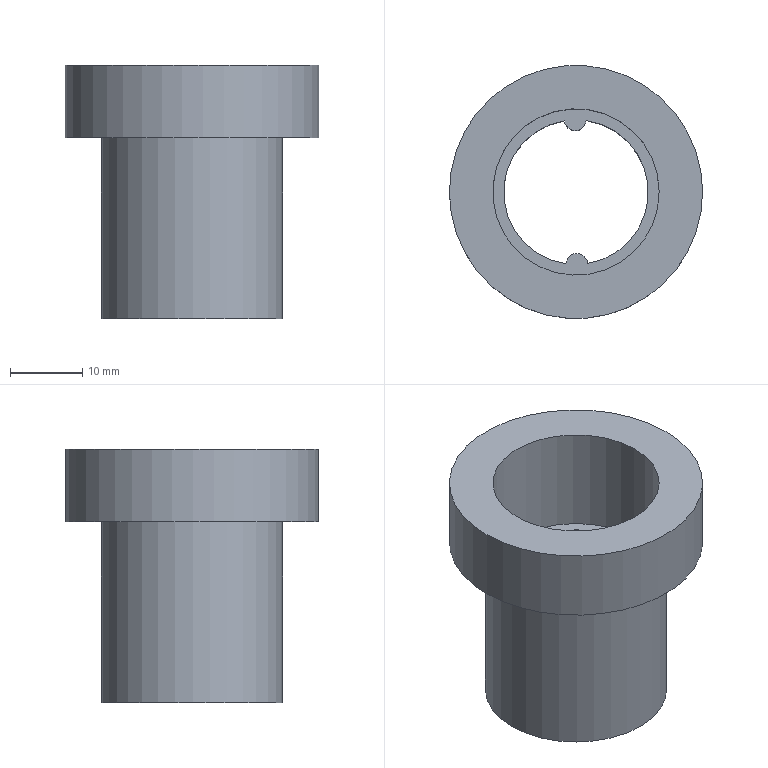Component | NX | BLANKDIE | 1 solid | 11 faces | box 35 x 35 x 35 mm | volume 9539 mm3 | cylinder 7 | plane 4 | commonest cylinder face diameters 20 x2 3 x2 25.025 x1 35 x1 23 x1
STEP:
#1=CARTESIAN_POINT('',(0.,0.,0.));
#2=DIRECTION('',(0.,0.,1.));
#3=DIRECTION('',(1.,0.,0.));
#4=AXIS2_PLACEMENT_3D('',#1,#2,#3);
#5=CARTESIAN_POINT('',(-1.603,-63.129,93.077));
#6=VERTEX_POINT('',#5);
#7=CARTESIAN_POINT('',(-1.603,-63.129,73.077));
#8=VERTEX_POINT('',#7);
#9=CARTESIAN_POINT('',(-1.603,-63.129,98.077));
#10=DIRECTION('',(0.,0.,-1.));
#11=VECTOR('',#10,1.);
#12=LINE('',#9,#11);
#13=CARTESIAN_POINT('',(-0.,-73.,98.077));
#14=DIRECTION('',(0.,0.,-1.));
#15=DIRECTION('',(-1.,-0.005818,0.));
#16=AXIS2_PLACEMENT_3D('',#13,#14,#15);
#17=CYLINDRICAL_SURFACE('',#16,10.);
#18=CARTESIAN_POINT('',(7.699,0.));
#19=DIRECTION('',(0.,1.));
#20=VECTOR('',#19,1.);
#21=LINE('',#18,#20);
#22=(GEOMETRIC_REPRESENTATION_CONTEXT(2)PARAMETRIC_REPRESENTATION_CONTEXT()REPRESENTATION_CONTEXT('',''));
#23=DEFINITIONAL_REPRESENTATION('',(#21),#22);
#24=PCURVE('',#17,#23);
#25=CARTESIAN_POINT('',(-0.1084,-63.001,98.077));
#26=DIRECTION('',(0.,0.,-1.));
#27=DIRECTION('',(-1.,-0.005818,0.));
#28=AXIS2_PLACEMENT_3D('',#25,#26,#27);
#29=CYLINDRICAL_SURFACE('',#28,1.5);
#30=CARTESIAN_POINT('',(6.203,0.));
#31=DIRECTION('',(0.,1.));
#32=VECTOR('',#31,1.);
#33=LINE('',#30,#32);
#34=(GEOMETRIC_REPRESENTATION_CONTEXT(2)PARAMETRIC_REPRESENTATION_CONTEXT()REPRESENTATION_CONTEXT('',''));
#35=DEFINITIONAL_REPRESENTATION('',(#33),#34);
#36=PCURVE('',#29,#35);
#37=SURFACE_CURVE('',#12,(#24,#36),.PCURVE_S1.);
#38=EDGE_CURVE('',#6,#8,#37,.T.);
#39=ORIENTED_EDGE('',*,*,#38,.T.);
#40=CARTESIAN_POINT('',(-1.388,-82.903,73.077));
#41=VERTEX_POINT('',#40);
#42=CARTESIAN_POINT('',(-0.,-73.,73.077));
#43=DIRECTION('',(0.,0.,1.));
#44=DIRECTION('',(1.,0.005818,0.));
#45=AXIS2_PLACEMENT_3D('',#42,#43,#44);
#46=CIRCLE('',#45,10.);
#47=CARTESIAN_POINT('',(9.425,25.));
#48=DIRECTION('',(-1.,0.));
#49=VECTOR('',#48,1.);
#50=LINE('',#47,#49);
#51=(GEOMETRIC_REPRESENTATION_CONTEXT(2)PARAMETRIC_REPRESENTATION_CONTEXT()REPRESENTATION_CONTEXT('',''));
#52=DEFINITIONAL_REPRESENTATION('',(#50),#51);
#53=PCURVE('',#17,#52);
#54=CARTESIAN_POINT('',(-0.03615,-69.667,73.077));
#55=DIRECTION('',(0.,0.,1.));
#56=DIRECTION('',(1.,0.005818,0.));
#57=AXIS2_PLACEMENT_3D('',#54,#55,#56);
#58=PLANE('',#57);
#59=CARTESIAN_POINT('',(0.01676,-3.333));
#60=DIRECTION('',(1.,-0.));
#61=AXIS2_PLACEMENT_2D('',#59,#60);
#62=CIRCLE('',#61,10.);
#63=(GEOMETRIC_REPRESENTATION_CONTEXT(2)PARAMETRIC_REPRESENTATION_CONTEXT()REPRESENTATION_CONTEXT('',''));
#64=DEFINITIONAL_REPRESENTATION('',(#62),#63);
#65=PCURVE('',#58,#64);
#66=SURFACE_CURVE('',#46,(#53,#65),.PCURVE_S1.);
#67=EDGE_CURVE('',#8,#41,#66,.T.);
#68=ORIENTED_EDGE('',*,*,#67,.T.);
#69=CARTESIAN_POINT('',(-1.388,-82.903,93.077));
#70=VERTEX_POINT('',#69);
#71=CARTESIAN_POINT('',(-1.388,-82.903,98.077));
#72=DIRECTION('',(0.,0.,-1.));
#73=VECTOR('',#72,1.);
#74=LINE('',#71,#73);
#75=CARTESIAN_POINT('',(4.858,0.));
#76=DIRECTION('',(0.,1.));
#77=VECTOR('',#76,1.);
#78=LINE('',#75,#77);
#79=(GEOMETRIC_REPRESENTATION_CONTEXT(2)PARAMETRIC_REPRESENTATION_CONTEXT()REPRESENTATION_CONTEXT('',''));
#80=DEFINITIONAL_REPRESENTATION('',(#78),#79);
#81=PCURVE('',#17,#80);
#82=CARTESIAN_POINT('',(0.1084,-82.999,98.077));
#83=DIRECTION('',(0.,0.,-1.));
#84=DIRECTION('',(-1.,-0.005818,0.));
#85=AXIS2_PLACEMENT_3D('',#82,#83,#84);
#86=CYLINDRICAL_SURFACE('',#85,1.5);
#87=CARTESIAN_POINT('',(0.07004,0.));
#88=DIRECTION('',(0.,1.));
#89=VECTOR('',#88,1.);
#90=LINE('',#87,#89);
#91=(GEOMETRIC_REPRESENTATION_CONTEXT(2)PARAMETRIC_REPRESENTATION_CONTEXT()REPRESENTATION_CONTEXT('',''));
#92=DEFINITIONAL_REPRESENTATION('',(#90),#91);
#93=PCURVE('',#86,#92);
#94=SURFACE_CURVE('',#74,(#81,#93),.PCURVE_S1.);
#95=EDGE_CURVE('',#70,#41,#94,.T.);
#96=ORIENTED_EDGE('',*,*,#95,.F.);
#97=CARTESIAN_POINT('',(-0.,-73.,93.077));
#98=DIRECTION('',(0.,0.,1.));
#99=DIRECTION('',(-1.,-0.005818,0.));
#100=AXIS2_PLACEMENT_3D('',#97,#98,#99);
#101=CIRCLE('',#100,10.);
#102=CARTESIAN_POINT('',(12.566,5.));
#103=DIRECTION('',(-1.,0.));
#104=VECTOR('',#103,1.);
#105=LINE('',#102,#104);
#106=(GEOMETRIC_REPRESENTATION_CONTEXT(2)PARAMETRIC_REPRESENTATION_CONTEXT()REPRESENTATION_CONTEXT('',''));
#107=DEFINITIONAL_REPRESENTATION('',(#105),#106);
#108=PCURVE('',#17,#107);
#109=CARTESIAN_POINT('',(-0.,-73.,93.077));
#110=DIRECTION('',(0.,0.,-1.));
#111=DIRECTION('',(-1.,-0.005818,0.));
#112=AXIS2_PLACEMENT_3D('',#109,#110,#111);
#113=PLANE('',#112);
#114=CARTESIAN_POINT('',(10.,0.));
#115=CARTESIAN_POINT('',(10.,-17.321));
#116=CARTESIAN_POINT('',(-5.,-8.66));
#117=CARTESIAN_POINT('',(-20.,-0.));
#118=CARTESIAN_POINT('',(-5.,8.66));
#119=CARTESIAN_POINT('',(10.,17.321));
#120=CARTESIAN_POINT('',(10.,0.));
#121=(BOUNDED_CURVE()B_SPLINE_CURVE(2,(#114,#115,#116,#117,#118,#119,#120),.UNSPECIFIED.,.T.,.F.)B_SPLINE_CURVE_WITH_KNOTS((1,2,2,2,2,1),(-2.094,0.,2.094,4.189,6.283,8.378),.UNSPECIFIED.)CURVE()GEOMETRIC_REPRESENTATION_ITEM()RATIONAL_B_SPLINE_CURVE((1.,0.5,1.,0.5,1.,0.5,1.))REPRESENTATION_ITEM(''));
#122=(GEOMETRIC_REPRESENTATION_CONTEXT(2)PARAMETRIC_REPRESENTATION_CONTEXT()REPRESENTATION_CONTEXT('',''));
#123=DEFINITIONAL_REPRESENTATION('',(#121),#122);
#124=PCURVE('',#113,#123);
#125=SURFACE_CURVE('',#101,(#108,#124),.PCURVE_S1.);
#126=EDGE_CURVE('',#6,#70,#125,.T.);
#127=ORIENTED_EDGE('',*,*,#126,.F.);
#128=EDGE_LOOP('',(#39,#68,#96,#127));
#129=FACE_BOUND('',#128,.F.);
#130=ADVANCED_FACE('',(#129),#17,.F.);
#131=CARTESIAN_POINT('',(1.388,-63.097,93.077));
#132=VERTEX_POINT('',#131);
#133=CARTESIAN_POINT('',(-0.1084,-63.001,93.077));
#134=DIRECTION('',(0.,0.,-1.));
#135=DIRECTION('',(-1.,-0.005818,0.));
#136=AXIS2_PLACEMENT_3D('',#133,#134,#135);
#137=CIRCLE('',#136,1.5);
#138=CARTESIAN_POINT('',(-0.,5.));
#139=DIRECTION('',(1.,0.));
#140=VECTOR('',#139,1.);
#141=LINE('',#138,#140);
#142=(GEOMETRIC_REPRESENTATION_CONTEXT(2)PARAMETRIC_REPRESENTATION_CONTEXT()REPRESENTATION_CONTEXT('',''));
#143=DEFINITIONAL_REPRESENTATION('',(#141),#142);
#144=PCURVE('',#29,#143);
#145=CARTESIAN_POINT('',(0.05027,10.));
#146=DIRECTION('',(1.,-0.));
#147=AXIS2_PLACEMENT_2D('',#145,#146);
#148=CIRCLE('',#147,1.5);
#149=(GEOMETRIC_REPRESENTATION_CONTEXT(2)PARAMETRIC_REPRESENTATION_CONTEXT()REPRESENTATION_CONTEXT('',''));
#150=DEFINITIONAL_REPRESENTATION('',(#148),#149);
#151=PCURVE('',#113,#150);
#152=SURFACE_CURVE('',#137,(#144,#151),.PCURVE_S1.);
#153=EDGE_CURVE('',#132,#6,#152,.T.);
#154=ORIENTED_EDGE('',*,*,#153,.T.);
#155=ORIENTED_EDGE('',*,*,#38,.T.);
#156=CARTESIAN_POINT('',(1.388,-63.097,73.077));
#157=VERTEX_POINT('',#156);
#158=CARTESIAN_POINT('',(-0.1084,-63.001,73.077));
#159=DIRECTION('',(0.,0.,-1.));
#160=DIRECTION('',(1.,0.005818,0.));
#161=AXIS2_PLACEMENT_3D('',#158,#159,#160);
#162=CIRCLE('',#161,1.5);
#163=CARTESIAN_POINT('',(3.142,25.));
#164=DIRECTION('',(1.,0.));
#165=VECTOR('',#164,1.);
#166=LINE('',#163,#165);
#167=(GEOMETRIC_REPRESENTATION_CONTEXT(2)PARAMETRIC_REPRESENTATION_CONTEXT()REPRESENTATION_CONTEXT('',''));
#168=DEFINITIONAL_REPRESENTATION('',(#166),#167);
#169=PCURVE('',#29,#168);
#170=CARTESIAN_POINT('',(1.466,6.667));
#171=CARTESIAN_POINT('',(1.466,4.069));
#172=CARTESIAN_POINT('',(-0.7835,5.368));
#173=CARTESIAN_POINT('',(-3.034,6.667));
#174=CARTESIAN_POINT('',(-0.7835,7.966));
#175=CARTESIAN_POINT('',(1.466,9.265));
#176=CARTESIAN_POINT('',(1.466,6.667));
#177=(BOUNDED_CURVE()B_SPLINE_CURVE(2,(#170,#171,#172,#173,#174,#175,#176),.UNSPECIFIED.,.T.,.F.)B_SPLINE_CURVE_WITH_KNOTS((1,2,2,2,2,1),(-2.094,0.,2.094,4.189,6.283,8.378),.UNSPECIFIED.)CURVE()GEOMETRIC_REPRESENTATION_ITEM()RATIONAL_B_SPLINE_CURVE((1.,0.5,1.,0.5,1.,0.5,1.))REPRESENTATION_ITEM(''));
#178=(GEOMETRIC_REPRESENTATION_CONTEXT(2)PARAMETRIC_REPRESENTATION_CONTEXT()REPRESENTATION_CONTEXT('',''));
#179=DEFINITIONAL_REPRESENTATION('',(#177),#178);
#180=PCURVE('',#58,#179);
#181=SURFACE_CURVE('',#162,(#169,#180),.PCURVE_S1.);
#182=EDGE_CURVE('',#157,#8,#181,.T.);
#183=ORIENTED_EDGE('',*,*,#182,.F.);
#184=CARTESIAN_POINT('',(1.388,-63.097,98.077));
#185=DIRECTION('',(0.,0.,-1.));
#186=VECTOR('',#185,1.);
#187=LINE('',#184,#186);
#188=CARTESIAN_POINT('',(3.212,0.));
#189=DIRECTION('',(0.,1.));
#190=VECTOR('',#189,1.);
#191=LINE('',#188,#190);
#192=(GEOMETRIC_REPRESENTATION_CONTEXT(2)PARAMETRIC_REPRESENTATION_CONTEXT()REPRESENTATION_CONTEXT('',''));
#193=DEFINITIONAL_REPRESENTATION('',(#191),#192);
#194=PCURVE('',#29,#193);
#195=CARTESIAN_POINT('',(-0.,-73.,98.077));
#196=DIRECTION('',(0.,0.,-1.));
#197=DIRECTION('',(-1.,-0.005818,0.));
#198=AXIS2_PLACEMENT_3D('',#195,#196,#197);
#199=CYLINDRICAL_SURFACE('',#198,10.);
#200=CARTESIAN_POINT('',(1.716,0.));
#201=DIRECTION('',(0.,1.));
#202=VECTOR('',#201,1.);
#203=LINE('',#200,#202);
#204=(GEOMETRIC_REPRESENTATION_CONTEXT(2)PARAMETRIC_REPRESENTATION_CONTEXT()REPRESENTATION_CONTEXT('',''));
#205=DEFINITIONAL_REPRESENTATION('',(#203),#204);
#206=PCURVE('',#199,#205);
#207=SURFACE_CURVE('',#187,(#194,#206),.PCURVE_S1.);
#208=EDGE_CURVE('',#132,#157,#207,.T.);
#209=ORIENTED_EDGE('',*,*,#208,.F.);
#210=EDGE_LOOP('',(#154,#155,#183,#209));
#211=FACE_BOUND('',#210,.T.);
#212=ADVANCED_FACE('',(#211),#29,.T.);
#213=CARTESIAN_POINT('',(1.603,-82.871,93.077));
#214=VERTEX_POINT('',#213);
#215=CARTESIAN_POINT('',(1.603,-82.871,73.077));
#216=VERTEX_POINT('',#215);
#217=CARTESIAN_POINT('',(1.603,-82.871,98.077));
#218=DIRECTION('',(0.,0.,-1.));
#219=VECTOR('',#218,1.);
#220=LINE('',#217,#219);
#221=CARTESIAN_POINT('',(4.557,0.));
#222=DIRECTION('',(0.,1.));
#223=VECTOR('',#222,1.);
#224=LINE('',#221,#223);
#225=(GEOMETRIC_REPRESENTATION_CONTEXT(2)PARAMETRIC_REPRESENTATION_CONTEXT()REPRESENTATION_CONTEXT('',''));
#226=DEFINITIONAL_REPRESENTATION('',(#224),#225);
#227=PCURVE('',#199,#226);
#228=CARTESIAN_POINT('',(3.061,0.));
#229=DIRECTION('',(0.,1.));
#230=VECTOR('',#229,1.);
#231=LINE('',#228,#230);
#232=(GEOMETRIC_REPRESENTATION_CONTEXT(2)PARAMETRIC_REPRESENTATION_CONTEXT()REPRESENTATION_CONTEXT('',''));
#233=DEFINITIONAL_REPRESENTATION('',(#231),#232);
#234=PCURVE('',#86,#233);
#235=SURFACE_CURVE('',#220,(#227,#234),.PCURVE_S1.);
#236=EDGE_CURVE('',#214,#216,#235,.T.);
#237=ORIENTED_EDGE('',*,*,#236,.T.);
#238=CARTESIAN_POINT('',(-0.,-73.,73.077));
#239=DIRECTION('',(0.,0.,1.));
#240=DIRECTION('',(1.,0.005818,0.));
#241=AXIS2_PLACEMENT_3D('',#238,#239,#240);
#242=CIRCLE('',#241,10.);
#243=CARTESIAN_POINT('',(9.425,25.));
#244=DIRECTION('',(-1.,0.));
#245=VECTOR('',#244,1.);
#246=LINE('',#243,#245);
#247=(GEOMETRIC_REPRESENTATION_CONTEXT(2)PARAMETRIC_REPRESENTATION_CONTEXT()REPRESENTATION_CONTEXT('',''));
#248=DEFINITIONAL_REPRESENTATION('',(#246),#247);
#249=PCURVE('',#199,#248);
#250=CARTESIAN_POINT('',(0.01676,-3.333));
#251=DIRECTION('',(1.,-0.));
#252=AXIS2_PLACEMENT_2D('',#250,#251);
#253=CIRCLE('',#252,10.);
#254=(GEOMETRIC_REPRESENTATION_CONTEXT(2)PARAMETRIC_REPRESENTATION_CONTEXT()REPRESENTATION_CONTEXT('',''));
#255=DEFINITIONAL_REPRESENTATION('',(#253),#254);
#256=PCURVE('',#58,#255);
#257=SURFACE_CURVE('',#242,(#249,#256),.PCURVE_S1.);
#258=EDGE_CURVE('',#216,#157,#257,.T.);
#259=ORIENTED_EDGE('',*,*,#258,.T.);
#260=ORIENTED_EDGE('',*,*,#208,.F.);
#261=CARTESIAN_POINT('',(-0.,-73.,93.077));
#262=DIRECTION('',(0.,0.,1.));
#263=DIRECTION('',(-1.,-0.005818,0.));
#264=AXIS2_PLACEMENT_3D('',#261,#262,#263);
#265=CIRCLE('',#264,10.);
#266=CARTESIAN_POINT('',(6.283,5.));
#267=DIRECTION('',(-1.,0.));
#268=VECTOR('',#267,1.);
#269=LINE('',#266,#268);
#270=(GEOMETRIC_REPRESENTATION_CONTEXT(2)PARAMETRIC_REPRESENTATION_CONTEXT()REPRESENTATION_CONTEXT('',''));
#271=DEFINITIONAL_REPRESENTATION('',(#269),#270);
#272=PCURVE('',#199,#271);
#273=CARTESIAN_POINT('',(10.,0.));
#274=CARTESIAN_POINT('',(10.,-17.321));
#275=CARTESIAN_POINT('',(-5.,-8.66));
#276=CARTESIAN_POINT('',(-20.,-0.));
#277=CARTESIAN_POINT('',(-5.,8.66));
#278=CARTESIAN_POINT('',(10.,17.321));
#279=CARTESIAN_POINT('',(10.,0.));
#280=(BOUNDED_CURVE()B_SPLINE_CURVE(2,(#273,#274,#275,#276,#277,#278,#279),.UNSPECIFIED.,.T.,.F.)B_SPLINE_CURVE_WITH_KNOTS((1,2,2,2,2,1),(-2.094,0.,2.094,4.189,6.283,8.378),.UNSPECIFIED.)CURVE()GEOMETRIC_REPRESENTATION_ITEM()RATIONAL_B_SPLINE_CURVE((1.,0.5,1.,0.5,1.,0.5,1.))REPRESENTATION_ITEM(''));
#281=(GEOMETRIC_REPRESENTATION_CONTEXT(2)PARAMETRIC_REPRESENTATION_CONTEXT()REPRESENTATION_CONTEXT('',''));
#282=DEFINITIONAL_REPRESENTATION('',(#280),#281);
#283=PCURVE('',#113,#282);
#284=SURFACE_CURVE('',#265,(#272,#283),.PCURVE_S1.);
#285=EDGE_CURVE('',#214,#132,#284,.T.);
#286=ORIENTED_EDGE('',*,*,#285,.F.);
#287=EDGE_LOOP('',(#237,#259,#260,#286));
#288=FACE_BOUND('',#287,.F.);
#289=ADVANCED_FACE('',(#288),#199,.F.);
#290=CARTESIAN_POINT('',(12.512,-72.927,98.077));
#291=VERTEX_POINT('',#290);
#292=CARTESIAN_POINT('',(-0.,-73.,98.077));
#293=DIRECTION('',(0.,0.,1.));
#294=DIRECTION('',(1.,0.005818,0.));
#295=AXIS2_PLACEMENT_3D('',#292,#293,#294);
#296=CIRCLE('',#295,12.512);
#297=CARTESIAN_POINT('',(-0.,-73.,98.077));
#298=DIRECTION('',(0.,0.,-1.));
#299=DIRECTION('',(-1.,-0.005818,0.));
#300=AXIS2_PLACEMENT_3D('',#297,#298,#299);
#301=CYLINDRICAL_SURFACE('',#300,12.512);
#302=CARTESIAN_POINT('',(9.425,0.));
#303=DIRECTION('',(-1.,0.));
#304=VECTOR('',#303,1.);
#305=LINE('',#302,#304);
#306=(GEOMETRIC_REPRESENTATION_CONTEXT(2)PARAMETRIC_REPRESENTATION_CONTEXT()REPRESENTATION_CONTEXT('',''));
#307=DEFINITIONAL_REPRESENTATION('',(#305),#306);
#308=PCURVE('',#301,#307);
#309=CARTESIAN_POINT('',(-0.,-73.,98.077));
#310=DIRECTION('',(0.,0.,1.));
#311=DIRECTION('',(1.,0.005818,0.));
#312=AXIS2_PLACEMENT_3D('',#309,#310,#311);
#313=PLANE('',#312);
#314=CARTESIAN_POINT('',(0.,0.));
#315=DIRECTION('',(1.,-0.));
#316=AXIS2_PLACEMENT_2D('',#314,#315);
#317=CIRCLE('',#316,12.512);
#318=(GEOMETRIC_REPRESENTATION_CONTEXT(2)PARAMETRIC_REPRESENTATION_CONTEXT()REPRESENTATION_CONTEXT('',''));
#319=DEFINITIONAL_REPRESENTATION('',(#317),#318);
#320=PCURVE('',#313,#319);
#321=SURFACE_CURVE('',#296,(#308,#320),.PCURVE_S1.);
#322=EDGE_CURVE('',#291,#291,#321,.T.);
#323=ORIENTED_EDGE('',*,*,#322,.F.);
#324=CARTESIAN_POINT('',(12.512,-72.927,73.077));
#325=VERTEX_POINT('',#324);
#326=CARTESIAN_POINT('',(12.512,-72.927,98.077));
#327=CARTESIAN_POINT('',(12.512,-72.927,73.077));
#328=B_SPLINE_CURVE_WITH_KNOTS('',1,(#326,#327),.UNSPECIFIED.,.F.,.F.,(2,2),(0.,25.),.PIECEWISE_BEZIER_KNOTS.);
#329=CARTESIAN_POINT('',(9.425,0.));
#330=DIRECTION('',(0.,1.));
#331=VECTOR('',#330,1.);
#332=LINE('',#329,#331);
#333=(GEOMETRIC_REPRESENTATION_CONTEXT(2)PARAMETRIC_REPRESENTATION_CONTEXT()REPRESENTATION_CONTEXT('',''));
#334=DEFINITIONAL_REPRESENTATION('',(#332),#333);
#335=PCURVE('',#301,#334);
#336=CARTESIAN_POINT('',(3.142,0.));
#337=DIRECTION('',(0.,1.));
#338=VECTOR('',#337,1.);
#339=LINE('',#336,#338);
#340=(GEOMETRIC_REPRESENTATION_CONTEXT(2)PARAMETRIC_REPRESENTATION_CONTEXT()REPRESENTATION_CONTEXT('',''));
#341=DEFINITIONAL_REPRESENTATION('',(#339),#340);
#342=PCURVE('',#301,#341);
#343=SEAM_CURVE('',#328,(#335,#342),.PCURVE_S1.);
#344=EDGE_CURVE('',#291,#325,#343,.T.);
#345=ORIENTED_EDGE('',*,*,#344,.T.);
#346=CARTESIAN_POINT('',(-0.,-73.,73.077));
#347=DIRECTION('',(0.,0.,1.));
#348=DIRECTION('',(1.,0.005818,0.));
#349=AXIS2_PLACEMENT_3D('',#346,#347,#348);
#350=CIRCLE('',#349,12.512);
#351=CARTESIAN_POINT('',(9.425,25.));
#352=DIRECTION('',(-1.,0.));
#353=VECTOR('',#352,1.);
#354=LINE('',#351,#353);
#355=(GEOMETRIC_REPRESENTATION_CONTEXT(2)PARAMETRIC_REPRESENTATION_CONTEXT()REPRESENTATION_CONTEXT('',''));
#356=DEFINITIONAL_REPRESENTATION('',(#354),#355);
#357=PCURVE('',#301,#356);
#358=CARTESIAN_POINT('',(0.01676,-3.333));
#359=DIRECTION('',(1.,-0.));
#360=AXIS2_PLACEMENT_2D('',#358,#359);
#361=CIRCLE('',#360,12.512);
#362=(GEOMETRIC_REPRESENTATION_CONTEXT(2)PARAMETRIC_REPRESENTATION_CONTEXT()REPRESENTATION_CONTEXT('',''));
#363=DEFINITIONAL_REPRESENTATION('',(#361),#362);
#364=PCURVE('',#58,#363);
#365=SURFACE_CURVE('',#350,(#357,#364),.PCURVE_S1.);
#366=EDGE_CURVE('',#325,#325,#365,.T.);
#367=ORIENTED_EDGE('',*,*,#366,.T.);
#368=ORIENTED_EDGE('',*,*,#344,.F.);
#369=EDGE_LOOP('',(#323,#345,#367,#368));
#370=FACE_BOUND('',#369,.T.);
#371=ADVANCED_FACE('',(#370),#301,.T.);
#372=CARTESIAN_POINT('',(0.1084,-82.999,93.077));
#373=DIRECTION('',(0.,0.,-1.));
#374=DIRECTION('',(-1.,-0.005818,0.));
#375=AXIS2_PLACEMENT_3D('',#372,#373,#374);
#376=CIRCLE('',#375,1.5);
#377=CARTESIAN_POINT('',(-0.,5.));
#378=DIRECTION('',(1.,0.));
#379=VECTOR('',#378,1.);
#380=LINE('',#377,#379);
#381=(GEOMETRIC_REPRESENTATION_CONTEXT(2)PARAMETRIC_REPRESENTATION_CONTEXT()REPRESENTATION_CONTEXT('',''));
#382=DEFINITIONAL_REPRESENTATION('',(#380),#381);
#383=PCURVE('',#86,#382);
#384=CARTESIAN_POINT('',(-0.05027,-10.));
#385=DIRECTION('',(1.,-0.));
#386=AXIS2_PLACEMENT_2D('',#384,#385);
#387=CIRCLE('',#386,1.5);
#388=(GEOMETRIC_REPRESENTATION_CONTEXT(2)PARAMETRIC_REPRESENTATION_CONTEXT()REPRESENTATION_CONTEXT('',''));
#389=DEFINITIONAL_REPRESENTATION('',(#387),#388);
#390=PCURVE('',#113,#389);
#391=SURFACE_CURVE('',#376,(#383,#390),.PCURVE_S1.);
#392=EDGE_CURVE('',#70,#214,#391,.T.);
#393=ORIENTED_EDGE('',*,*,#392,.T.);
#394=ORIENTED_EDGE('',*,*,#236,.T.);
#395=CARTESIAN_POINT('',(0.1084,-82.999,73.077));
#396=DIRECTION('',(0.,0.,-1.));
#397=DIRECTION('',(1.,0.005818,0.));
#398=AXIS2_PLACEMENT_3D('',#395,#396,#397);
#399=CIRCLE('',#398,1.5);
#400=CARTESIAN_POINT('',(-3.142,25.));
#401=DIRECTION('',(1.,0.));
#402=VECTOR('',#401,1.);
#403=LINE('',#400,#402);
#404=(GEOMETRIC_REPRESENTATION_CONTEXT(2)PARAMETRIC_REPRESENTATION_CONTEXT()REPRESENTATION_CONTEXT('',''));
#405=DEFINITIONAL_REPRESENTATION('',(#403),#404);
#406=PCURVE('',#86,#405);
#407=CARTESIAN_POINT('',(1.567,-13.333));
#408=CARTESIAN_POINT('',(1.567,-15.931));
#409=CARTESIAN_POINT('',(-0.683,-14.632));
#410=CARTESIAN_POINT('',(-2.933,-13.333));
#411=CARTESIAN_POINT('',(-0.683,-12.034));
#412=CARTESIAN_POINT('',(1.567,-10.735));
#413=CARTESIAN_POINT('',(1.567,-13.333));
#414=(BOUNDED_CURVE()B_SPLINE_CURVE(2,(#407,#408,#409,#410,#411,#412,#413),.UNSPECIFIED.,.T.,.F.)B_SPLINE_CURVE_WITH_KNOTS((1,2,2,2,2,1),(-2.094,0.,2.094,4.189,6.283,8.378),.UNSPECIFIED.)CURVE()GEOMETRIC_REPRESENTATION_ITEM()RATIONAL_B_SPLINE_CURVE((1.,0.5,1.,0.5,1.,0.5,1.))REPRESENTATION_ITEM(''));
#415=(GEOMETRIC_REPRESENTATION_CONTEXT(2)PARAMETRIC_REPRESENTATION_CONTEXT()REPRESENTATION_CONTEXT('',''));
#416=DEFINITIONAL_REPRESENTATION('',(#414),#415);
#417=PCURVE('',#58,#416);
#418=SURFACE_CURVE('',#399,(#406,#417),.PCURVE_S1.);
#419=EDGE_CURVE('',#41,#216,#418,.T.);
#420=ORIENTED_EDGE('',*,*,#419,.F.);
#421=ORIENTED_EDGE('',*,*,#95,.F.);
#422=EDGE_LOOP('',(#393,#394,#420,#421));
#423=FACE_BOUND('',#422,.T.);
#424=ADVANCED_FACE('',(#423),#86,.T.);
#425=ORIENTED_EDGE('',*,*,#366,.F.);
#426=EDGE_LOOP('',(#425));
#427=FACE_BOUND('',#426,.T.);
#428=ORIENTED_EDGE('',*,*,#67,.T.);
#429=ORIENTED_EDGE('',*,*,#419,.T.);
#430=ORIENTED_EDGE('',*,*,#258,.T.);
#431=ORIENTED_EDGE('',*,*,#182,.T.);
#432=EDGE_LOOP('',(#428,#429,#430,#431));
#433=FACE_BOUND('',#432,.T.);
#434=ADVANCED_FACE('',(#427,#433),#58,.F.);
#435=CARTESIAN_POINT('',(17.5,-72.898,98.077));
#436=VERTEX_POINT('',#435);
#437=CARTESIAN_POINT('',(-0.,-73.,98.077));
#438=DIRECTION('',(0.,0.,1.));
#439=DIRECTION('',(1.,0.005818,0.));
#440=AXIS2_PLACEMENT_3D('',#437,#438,#439);
#441=CIRCLE('',#440,17.5);
#442=CARTESIAN_POINT('',(0.,0.));
#443=DIRECTION('',(1.,-0.));
#444=AXIS2_PLACEMENT_2D('',#442,#443);
#445=CIRCLE('',#444,17.5);
#446=(GEOMETRIC_REPRESENTATION_CONTEXT(2)PARAMETRIC_REPRESENTATION_CONTEXT()REPRESENTATION_CONTEXT('',''));
#447=DEFINITIONAL_REPRESENTATION('',(#445),#446);
#448=PCURVE('',#313,#447);
#449=CARTESIAN_POINT('',(-0.,-73.,108.077));
#450=DIRECTION('',(0.,0.,-1.));
#451=DIRECTION('',(-1.,-0.005818,0.));
#452=AXIS2_PLACEMENT_3D('',#449,#450,#451);
#453=CYLINDRICAL_SURFACE('',#452,17.5);
#454=CARTESIAN_POINT('',(9.425,10.));
#455=DIRECTION('',(-1.,0.));
#456=VECTOR('',#455,1.);
#457=LINE('',#454,#456);
#458=(GEOMETRIC_REPRESENTATION_CONTEXT(2)PARAMETRIC_REPRESENTATION_CONTEXT()REPRESENTATION_CONTEXT('',''));
#459=DEFINITIONAL_REPRESENTATION('',(#457),#458);
#460=PCURVE('',#453,#459);
#461=SURFACE_CURVE('',#441,(#448,#460),.PCURVE_S1.);
#462=EDGE_CURVE('',#436,#436,#461,.T.);
#463=ORIENTED_EDGE('',*,*,#462,.F.);
#464=EDGE_LOOP('',(#463));
#465=FACE_BOUND('',#464,.T.);
#466=ORIENTED_EDGE('',*,*,#322,.T.);
#467=EDGE_LOOP('',(#466));
#468=FACE_BOUND('',#467,.T.);
#469=ADVANCED_FACE('',(#465,#468),#313,.F.);
#470=CARTESIAN_POINT('',(17.5,-72.898,108.077));
#471=VERTEX_POINT('',#470);
#472=CARTESIAN_POINT('',(-0.,-73.,108.077));
#473=DIRECTION('',(0.,0.,1.));
#474=DIRECTION('',(1.,0.005818,0.));
#475=AXIS2_PLACEMENT_3D('',#472,#473,#474);
#476=CIRCLE('',#475,17.5);
#477=CARTESIAN_POINT('',(9.425,0.));
#478=DIRECTION('',(-1.,0.));
#479=VECTOR('',#478,1.);
#480=LINE('',#477,#479);
#481=(GEOMETRIC_REPRESENTATION_CONTEXT(2)PARAMETRIC_REPRESENTATION_CONTEXT()REPRESENTATION_CONTEXT('',''));
#482=DEFINITIONAL_REPRESENTATION('',(#480),#481);
#483=PCURVE('',#453,#482);
#484=CARTESIAN_POINT('',(-0.,-73.,108.077));
#485=DIRECTION('',(0.,0.,1.));
#486=DIRECTION('',(1.,0.005818,0.));
#487=AXIS2_PLACEMENT_3D('',#484,#485,#486);
#488=PLANE('',#487);
#489=CARTESIAN_POINT('',(0.,0.));
#490=DIRECTION('',(1.,-0.));
#491=AXIS2_PLACEMENT_2D('',#489,#490);
#492=CIRCLE('',#491,17.5);
#493=(GEOMETRIC_REPRESENTATION_CONTEXT(2)PARAMETRIC_REPRESENTATION_CONTEXT()REPRESENTATION_CONTEXT('',''));
#494=DEFINITIONAL_REPRESENTATION('',(#492),#493);
#495=PCURVE('',#488,#494);
#496=SURFACE_CURVE('',#476,(#483,#495),.PCURVE_S1.);
#497=EDGE_CURVE('',#471,#471,#496,.T.);
#498=ORIENTED_EDGE('',*,*,#497,.F.);
#499=CARTESIAN_POINT('',(17.5,-72.898,108.077));
#500=CARTESIAN_POINT('',(17.5,-72.898,98.077));
#501=B_SPLINE_CURVE_WITH_KNOTS('',1,(#499,#500),.UNSPECIFIED.,.F.,.F.,(2,2),(0.,10.),.PIECEWISE_BEZIER_KNOTS.);
#502=CARTESIAN_POINT('',(9.425,0.));
#503=DIRECTION('',(0.,1.));
#504=VECTOR('',#503,1.);
#505=LINE('',#502,#504);
#506=(GEOMETRIC_REPRESENTATION_CONTEXT(2)PARAMETRIC_REPRESENTATION_CONTEXT()REPRESENTATION_CONTEXT('',''));
#507=DEFINITIONAL_REPRESENTATION('',(#505),#506);
#508=PCURVE('',#453,#507);
#509=CARTESIAN_POINT('',(3.142,0.));
#510=DIRECTION('',(0.,1.));
#511=VECTOR('',#510,1.);
#512=LINE('',#509,#511);
#513=(GEOMETRIC_REPRESENTATION_CONTEXT(2)PARAMETRIC_REPRESENTATION_CONTEXT()REPRESENTATION_CONTEXT('',''));
#514=DEFINITIONAL_REPRESENTATION('',(#512),#513);
#515=PCURVE('',#453,#514);
#516=SEAM_CURVE('',#501,(#508,#515),.PCURVE_S1.);
#517=EDGE_CURVE('',#471,#436,#516,.T.);
#518=ORIENTED_EDGE('',*,*,#517,.T.);
#519=ORIENTED_EDGE('',*,*,#462,.T.);
#520=ORIENTED_EDGE('',*,*,#517,.F.);
#521=EDGE_LOOP('',(#498,#518,#519,#520));
#522=FACE_BOUND('',#521,.T.);
#523=ADVANCED_FACE('',(#522),#453,.T.);
#524=CARTESIAN_POINT('',(11.5,-72.933,108.077));
#525=VERTEX_POINT('',#524);
#526=CARTESIAN_POINT('',(-0.,-73.,108.077));
#527=DIRECTION('',(0.,0.,-1.));
#528=DIRECTION('',(1.,0.005818,0.));
#529=AXIS2_PLACEMENT_3D('',#526,#527,#528);
#530=CIRCLE('',#529,11.5);
#531=CARTESIAN_POINT('',(11.5,-0.));
#532=CARTESIAN_POINT('',(11.5,-19.919));
#533=CARTESIAN_POINT('',(-5.75,-9.959));
#534=CARTESIAN_POINT('',(-23.,-0.));
#535=CARTESIAN_POINT('',(-5.75,9.959));
#536=CARTESIAN_POINT('',(11.5,19.919));
#537=CARTESIAN_POINT('',(11.5,-0.));
#538=(BOUNDED_CURVE()B_SPLINE_CURVE(2,(#531,#532,#533,#534,#535,#536,#537),.UNSPECIFIED.,.T.,.F.)B_SPLINE_CURVE_WITH_KNOTS((1,2,2,2,2,1),(-2.094,0.,2.094,4.189,6.283,8.378),.UNSPECIFIED.)CURVE()GEOMETRIC_REPRESENTATION_ITEM()RATIONAL_B_SPLINE_CURVE((1.,0.5,1.,0.5,1.,0.5,1.))REPRESENTATION_ITEM(''));
#539=(GEOMETRIC_REPRESENTATION_CONTEXT(2)PARAMETRIC_REPRESENTATION_CONTEXT()REPRESENTATION_CONTEXT('',''));
#540=DEFINITIONAL_REPRESENTATION('',(#538),#539);
#541=PCURVE('',#488,#540);
#542=CARTESIAN_POINT('',(-0.,-73.,93.077));
#543=DIRECTION('',(0.,0.,1.));
#544=DIRECTION('',(1.,0.005818,0.));
#545=AXIS2_PLACEMENT_3D('',#542,#543,#544);
#546=CYLINDRICAL_SURFACE('',#545,11.5);
#547=CARTESIAN_POINT('',(6.283,15.));
#548=DIRECTION('',(-1.,0.));
#549=VECTOR('',#548,1.);
#550=LINE('',#547,#549);
#551=(GEOMETRIC_REPRESENTATION_CONTEXT(2)PARAMETRIC_REPRESENTATION_CONTEXT()REPRESENTATION_CONTEXT('',''));
#552=DEFINITIONAL_REPRESENTATION('',(#550),#551);
#553=PCURVE('',#546,#552);
#554=SURFACE_CURVE('',#530,(#541,#553),.PCURVE_S1.);
#555=EDGE_CURVE('',#525,#525,#554,.T.);
#556=ORIENTED_EDGE('',*,*,#555,.T.);
#557=EDGE_LOOP('',(#556));
#558=FACE_BOUND('',#557,.T.);
#559=ORIENTED_EDGE('',*,*,#497,.T.);
#560=EDGE_LOOP('',(#559));
#561=FACE_BOUND('',#560,.T.);
#562=ADVANCED_FACE('',(#558,#561),#488,.T.);
#563=CARTESIAN_POINT('',(11.5,-72.933,93.077));
#564=VERTEX_POINT('',#563);
#565=CARTESIAN_POINT('',(-0.,-73.,93.077));
#566=DIRECTION('',(0.,0.,1.));
#567=DIRECTION('',(1.,0.005818,0.));
#568=AXIS2_PLACEMENT_3D('',#565,#566,#567);
#569=CIRCLE('',#568,11.5);
#570=CARTESIAN_POINT('',(0.,0.));
#571=DIRECTION('',(1.,0.));
#572=VECTOR('',#571,1.);
#573=LINE('',#570,#572);
#574=(GEOMETRIC_REPRESENTATION_CONTEXT(2)PARAMETRIC_REPRESENTATION_CONTEXT()REPRESENTATION_CONTEXT('',''));
#575=DEFINITIONAL_REPRESENTATION('',(#573),#574);
#576=PCURVE('',#546,#575);
#577=CARTESIAN_POINT('',(-11.5,-0.));
#578=CARTESIAN_POINT('',(-11.5,19.919));
#579=CARTESIAN_POINT('',(5.75,9.959));
#580=CARTESIAN_POINT('',(23.,0.));
#581=CARTESIAN_POINT('',(5.75,-9.959));
#582=CARTESIAN_POINT('',(-11.5,-19.919));
#583=CARTESIAN_POINT('',(-11.5,-0.));
#584=(BOUNDED_CURVE()B_SPLINE_CURVE(2,(#577,#578,#579,#580,#581,#582,#583),.UNSPECIFIED.,.T.,.F.)B_SPLINE_CURVE_WITH_KNOTS((1,2,2,2,2,1),(-2.094,0.,2.094,4.189,6.283,8.378),.UNSPECIFIED.)CURVE()GEOMETRIC_REPRESENTATION_ITEM()RATIONAL_B_SPLINE_CURVE((1.,0.5,1.,0.5,1.,0.5,1.))REPRESENTATION_ITEM(''));
#585=(GEOMETRIC_REPRESENTATION_CONTEXT(2)PARAMETRIC_REPRESENTATION_CONTEXT()REPRESENTATION_CONTEXT('',''));
#586=DEFINITIONAL_REPRESENTATION('',(#584),#585);
#587=PCURVE('',#113,#586);
#588=SURFACE_CURVE('',#569,(#576,#587),.PCURVE_S1.);
#589=EDGE_CURVE('',#564,#564,#588,.T.);
#590=ORIENTED_EDGE('',*,*,#589,.T.);
#591=CARTESIAN_POINT('',(11.5,-72.933,93.077));
#592=CARTESIAN_POINT('',(11.5,-72.933,108.077));
#593=B_SPLINE_CURVE_WITH_KNOTS('',1,(#591,#592),.UNSPECIFIED.,.F.,.F.,(2,2),(0.,15.),.PIECEWISE_BEZIER_KNOTS.);
#594=CARTESIAN_POINT('',(6.283,0.));
#595=DIRECTION('',(0.,1.));
#596=VECTOR('',#595,1.);
#597=LINE('',#594,#596);
#598=(GEOMETRIC_REPRESENTATION_CONTEXT(2)PARAMETRIC_REPRESENTATION_CONTEXT()REPRESENTATION_CONTEXT('',''));
#599=DEFINITIONAL_REPRESENTATION('',(#597),#598);
#600=PCURVE('',#546,#599);
#601=CARTESIAN_POINT('',(0.,0.));
#602=DIRECTION('',(0.,1.));
#603=VECTOR('',#602,1.);
#604=LINE('',#601,#603);
#605=(GEOMETRIC_REPRESENTATION_CONTEXT(2)PARAMETRIC_REPRESENTATION_CONTEXT()REPRESENTATION_CONTEXT('',''));
#606=DEFINITIONAL_REPRESENTATION('',(#604),#605);
#607=PCURVE('',#546,#606);
#608=SEAM_CURVE('',#593,(#600,#607),.PCURVE_S1.);
#609=EDGE_CURVE('',#564,#525,#608,.T.);
#610=ORIENTED_EDGE('',*,*,#609,.T.);
#611=ORIENTED_EDGE('',*,*,#555,.T.);
#612=ORIENTED_EDGE('',*,*,#609,.F.);
#613=EDGE_LOOP('',(#590,#610,#611,#612));
#614=FACE_BOUND('',#613,.F.);
#615=ADVANCED_FACE('',(#614),#546,.F.);
#616=ORIENTED_EDGE('',*,*,#126,.F.);
#617=ORIENTED_EDGE('',*,*,#153,.F.);
#618=ORIENTED_EDGE('',*,*,#285,.F.);
#619=ORIENTED_EDGE('',*,*,#392,.F.);
#620=EDGE_LOOP('',(#616,#617,#618,#619));
#621=FACE_BOUND('',#620,.T.);
#622=ORIENTED_EDGE('',*,*,#589,.T.);
#623=EDGE_LOOP('',(#622));
#624=FACE_BOUND('',#623,.T.);
#625=ADVANCED_FACE('',(#621,#624),#113,.F.);
#626=CLOSED_SHELL('',(#130,#212,#289,#371,#424,#434,#469,#523,#562,#615,#625));
#627=MANIFOLD_SOLID_BREP('',#626);
#628=(LENGTH_UNIT()NAMED_UNIT(*)SI_UNIT(.MILLI.,.METRE.));
#629=UNCERTAINTY_MEASURE_WITH_UNIT(LENGTH_MEASURE(0.000002),#628,'','');
#630=(NAMED_UNIT(*)PLANE_ANGLE_UNIT()SI_UNIT($,.RADIAN.));
#631=(NAMED_UNIT(*)SI_UNIT($,.STERADIAN.)SOLID_ANGLE_UNIT());
#632=(GEOMETRIC_REPRESENTATION_CONTEXT(3)GLOBAL_UNCERTAINTY_ASSIGNED_CONTEXT((#629))GLOBAL_UNIT_ASSIGNED_CONTEXT((#628,#630,#631))REPRESENTATION_CONTEXT('',''));
#633=ADVANCED_BREP_SHAPE_REPRESENTATION('',(#4,#627),#632);